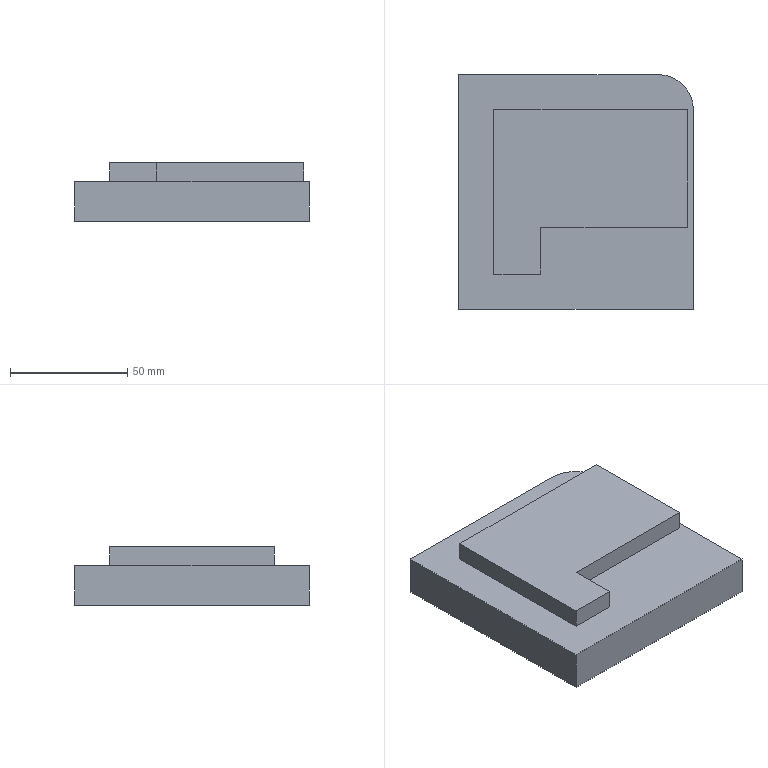CAM job | NX | mm | 3-axis | 1 set-up | 2 operations | part box 100 x 100 x 25
set-up 1
1. Planar Milling | Mill Mill5 D12 | PLANAR_MILL | path 8631.432 mm | 3.438 min
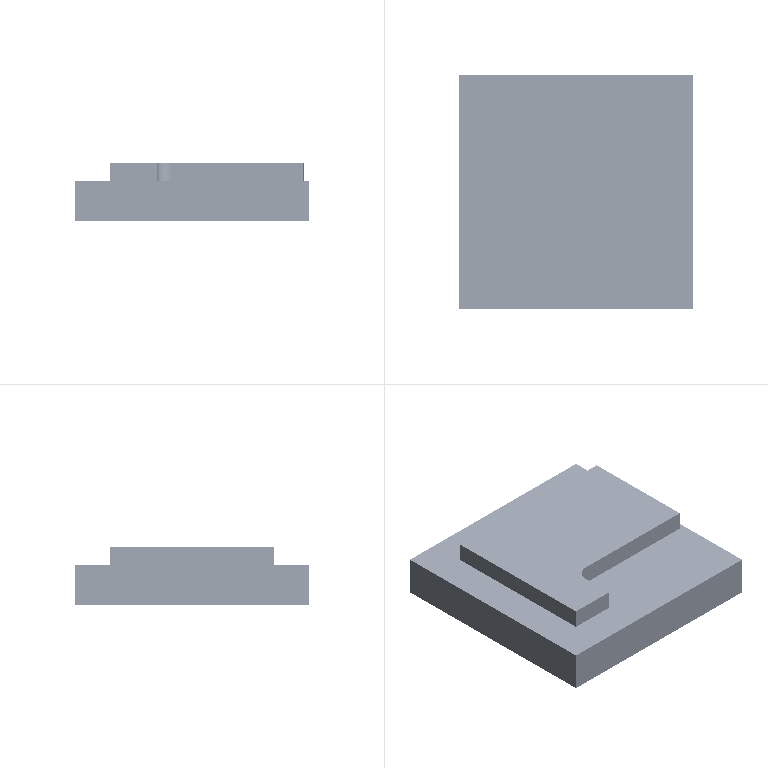2. Planar Milling | Mill Mill5 D12 | PLANAR_MILL_COPY | path 8632.765 mm | 3.438 min